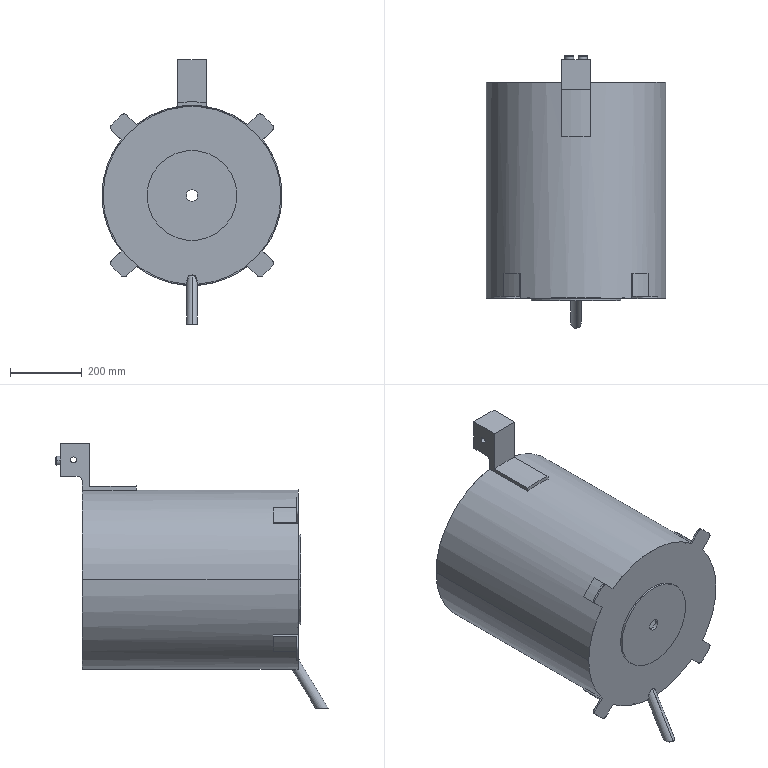Component | SolidWorks | Housing-2 | 1 solid | 78 faces | volume 4597457 mm3 | cylinder 42 | plane 32 | torus 4 | commonest cylinder face diameters 20 x10 30 x5 25 x4 594 x4 510 x4 494 x3 500 x3 16 x2